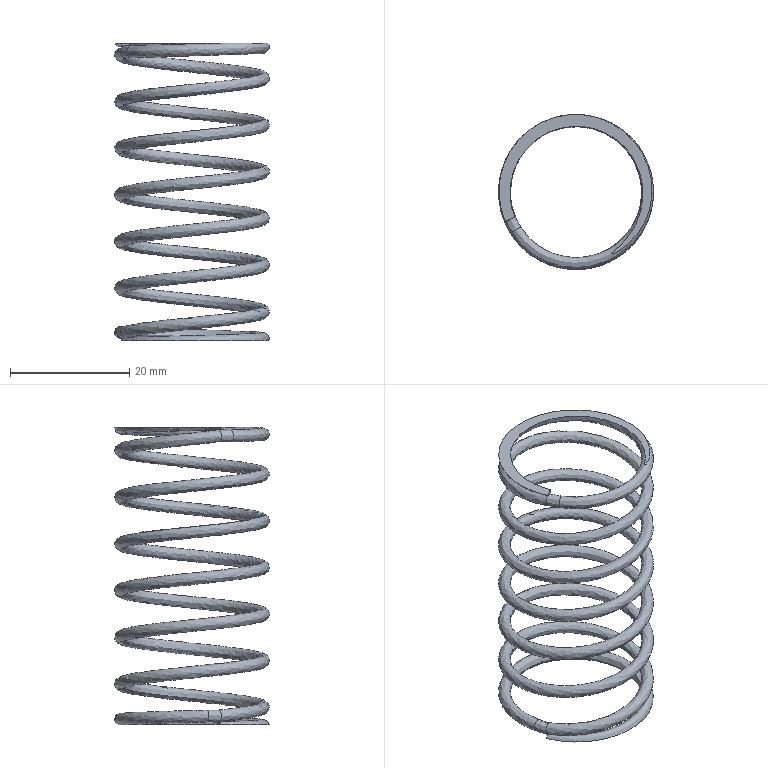Component | NX | SPRING_CYLINDER_COMPRESSION_1 | 1 solid | 9 faces | volume 1757 mm3 | spline 5 | plane 4